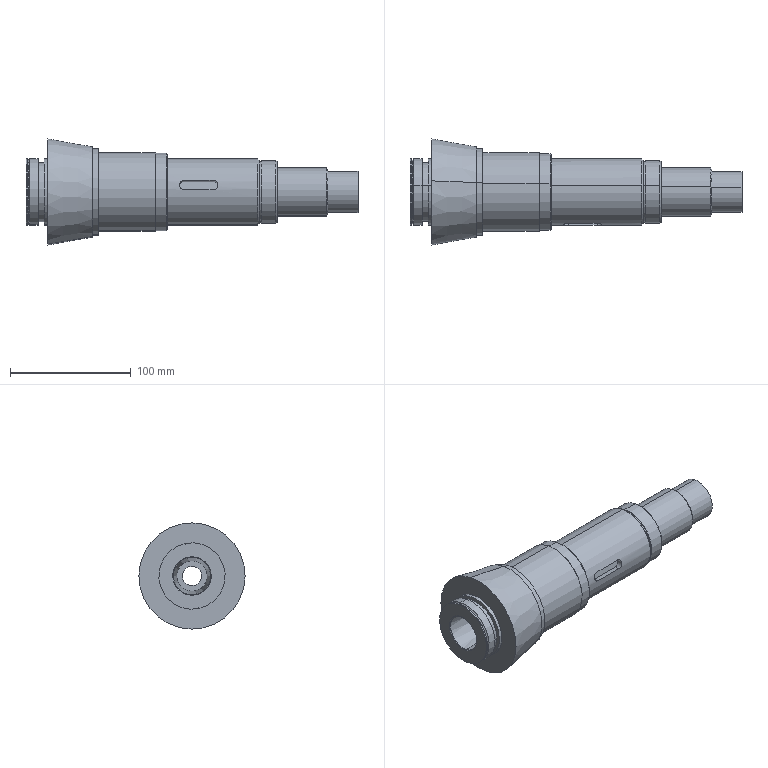Component | SolidWorks | 27Spindle-1 | 1 solid | 75 faces | box 275 x 88 x 88 mm | volume 621740 mm3 | cylinder 33 | plane 21 | cone 17 | torus 4 | commonest cylinder face diameters 55 x8 64 x3 16 x2 28 x2 34 x2 40 x2 52 x2 50 x2
build123d program:
from build123d import *
from OCP.BRepFilletAPI import BRepFilletAPI_MakeChamfer

# Parameters (mm, degrees)
SKETCH27_R           = 27.5
BOSS_EXTRUDE15_DEPTH = 10
SKETCH28_R           = 24.5
BOSS_EXTRUDE16_DEPTH = 5
SKETCH29_R           = 27.5
BOSS_EXTRUDE17_DEPTH = 3
SKETCH30_R           = 44
BOSS_EXTRUDE18_DEPTH = 37
BOSS_EXTRUDE18_TAPER = 10
SKETCH31_R           = 36
BOSS_EXTRUDE19_DEPTH = 5
SKETCH32_R           = 32.5
BOSS_EXTRUDE20_DEPTH = 47
SKETCH33_R           = 32
BOSS_EXTRUDE21_DEPTH = 10
BOSS_EXTRUDE22_START = -57
SKETCH34_R           = 27.5
BOSS_EXTRUDE22_DEPTH = 133
SKETCH35_R           = 25
BOSS_EXTRUDE23_DEPTH = 2
SKETCH36_R           = 26
BOSS_EXTRUDE24_DEPTH = 13
SKETCH37_R           = 20
BOSS_EXTRUDE25_DEPTH = 42
BOSS_EXTRUDE26_START = -250
SKETCH38_R           = 17
BOSS_EXTRUDE26_DEPTH = 275
SKETCH43_R           = 8
CUT_EXTRUDE3_DEPTH   = 180.154
CHAMFER1_SIZE        = 0.5
CHAMFER1_SIZE2       = 0.5164
CHAMFER2_SIZE        = 1
CUT_SWEEP1_PROFILE_R = 1
CUT_EXTRUDE4_DEPTH   = 4
CUT_EXTRUDE5_START   = -27.5
CUT_EXTRUDE5_DEPTH   = 5


with BuildPart() as part:
    # Sketch27 → Boss-Extrude15 (new body)
    with BuildSketch(Plane(origin=(0, 0, 0), x_dir=(0, 0, -1), z_dir=(1, 0, 0))):
        Circle(SKETCH27_R)
    extrude(amount=BOSS_EXTRUDE15_DEPTH)

    # Sketch28 → Boss-Extrude16 (add)
    with BuildSketch(Plane(origin=(10, 0, 0), x_dir=(0, 0, -1), z_dir=(1, 0, 0))):
        Circle(SKETCH28_R)
    extrude(amount=BOSS_EXTRUDE16_DEPTH)

    # Sketch29 → Boss-Extrude17 (add)
    with BuildSketch(Plane(origin=(15, 0, 0), x_dir=(0, 0, -1), z_dir=(1, 0, 0))):
        Circle(SKETCH29_R)
    extrude(amount=BOSS_EXTRUDE17_DEPTH)

    # Sketch30 → Boss-Extrude18 (add)
    with BuildSketch(Plane(origin=(18, 0, 0), x_dir=(0, 0, -1), z_dir=(1, 0, 0))):
        Circle(SKETCH30_R)
    extrude(amount=BOSS_EXTRUDE18_DEPTH, taper=BOSS_EXTRUDE18_TAPER)

    # Sketch31 → Boss-Extrude19 (add)
    with BuildSketch(Plane(origin=(55, 0, 0), x_dir=(0, 0, -1), z_dir=(1, 0, 0))):
        Circle(SKETCH31_R)
    extrude(amount=BOSS_EXTRUDE19_DEPTH)

    # Sketch32 → Boss-Extrude20 (add)
    with BuildSketch(Plane(origin=(60, 0, 0), x_dir=(0, 0, -1), z_dir=(1, 0, 0))):
        Circle(SKETCH32_R)
    extrude(amount=BOSS_EXTRUDE20_DEPTH)

    # Sketch33 → Boss-Extrude21 (add)
    with BuildSketch(Plane(origin=(107, 0, 0), x_dir=(0, 0, -1), z_dir=(1, 0, 0))):
        Circle(SKETCH33_R)
    extrude(amount=BOSS_EXTRUDE21_DEPTH)

    # Sketch34 → Boss-Extrude22 (add)
    with BuildSketch(Plane(origin=(117, 0, 0), x_dir=(0, 0, -1), z_dir=(1, 0, 0)).offset(BOSS_EXTRUDE22_START)):
        Circle(SKETCH34_R)
    extrude(amount=BOSS_EXTRUDE22_DEPTH)

    # Sketch35 → Boss-Extrude23 (add)
    with BuildSketch(Plane(origin=(193, 0, 0), x_dir=(0, 0, -1), z_dir=(1, 0, 0))):
        Circle(SKETCH35_R)
    extrude(amount=BOSS_EXTRUDE23_DEPTH)

    # Sketch36 → Boss-Extrude24 (add)
    with BuildSketch(Plane(origin=(195, 0, 0), x_dir=(0, 0, -1), z_dir=(1, 0, 0))):
        with Locations(Location((0, 0, 0), (0, 0, 180))):
            Circle(SKETCH36_R)
    extrude(amount=BOSS_EXTRUDE24_DEPTH)

    # Sketch37 → Boss-Extrude25 (add)
    with BuildSketch(Plane(origin=(208, 0, 0), x_dir=(0, 0, -1), z_dir=(1, 0, 0))):
        with Locations(Location((0, 0, 0), (0, 0, 180))):
            Circle(SKETCH37_R)
    extrude(amount=BOSS_EXTRUDE25_DEPTH)

    # Sketch38 → Boss-Extrude26 (add)
    with BuildSketch(Plane(origin=(250, 0, 0), x_dir=(0, 0, -1), z_dir=(1, 0, 0)).offset(BOSS_EXTRUDE26_START)):
        Circle(SKETCH38_R)
    extrude(amount=BOSS_EXTRUDE26_DEPTH)

    # Sketch42 → Cut-Revolve1 (revolve, cut)
    with BuildSketch(Plane(origin=(0, 0, 0), x_dir=(1, 0, 0), z_dir=(0, 1, 0)), mode=Mode.PRIVATE) as cut_revolve1_sk:
        Polygon((0, 0), (0, 15.5), (92, 12.625), (92, 14), (107, 14), (107, 0), align=None)
    revolve(cut_revolve1_sk.sketch.rotate(Axis((-73.512, 0, 0), (1, 0, 0)), 180), axis=Axis((-73.512, 0, 0), (1, 0, 0)), mode=Mode.SUBTRACT)

    # Sketch43 → Cut-Extrude3 (cut, through all)
    with BuildSketch(Plane.ZY.offset(-107)):
        Circle(SKETCH43_R)
    extrude(amount=-CUT_EXTRUDE3_DEPTH, mode=Mode.SUBTRACT)

    # Chamfer1: one chamfer whose edges measure the first distance from different faces: ONE call of the kernel's chamfer builder (chamfer() names one face for all edges)
    chamfer1_edges_1 = [part.edges().sort_by_distance(p)[0] for p in [
        (0, 0, -15.5),
    ]]
    chamfer1_side_1 = [part.faces().sort_by_distance(p)[0] for p in [
        (0, 0, 26.722),
    ]]
    chamfer1_edges_2 = [part.edges().sort_by_distance(p)[0] for p in [
        (275, 0, -8),
    ]]
    chamfer1 = BRepFilletAPI_MakeChamfer(part.part.solid().wrapped)
    for e in chamfer1_edges_1:
        chamfer1.Add(CHAMFER1_SIZE, CHAMFER1_SIZE2, e.wrapped, chamfer1_side_1[0].wrapped)  # the first distance lies on this face
    for e in chamfer1_edges_2:
        chamfer1.Add(CHAMFER1_SIZE, e.wrapped)
    add(Compound.cast(chamfer1.Shape()), mode=Mode.REPLACE)

    # Chamfer2
    chamfer2_edges = [part.edges().sort_by_distance(p)[0] for p in [
        (117, 0, 32),
        (193, 0, 27.5),
        (208, 0, -26),
        (250, 0, -20),
    ]]
    chamfer(chamfer2_edges, length=CHAMFER2_SIZE)

    # Cut-Sweep1: sweep along a path in Sketch44
    with BuildLine(Plane.ZY.offset(-2)) as cut_sweep1_path:
        CenterArc((0, 0), 27.5, 0, 360)
    # Cut-Sweep1 profile (on start of the path) → Cut-Sweep1 (sweep, cut)
    with BuildSketch(Plane(origin=(2, 0, 27.5), x_dir=(0, 0, 1), z_dir=(0, 1, 0))):
        Circle(CUT_SWEEP1_PROFILE_R)
    sweep(path=cut_sweep1_path.line, mode=Mode.SUBTRACT)

    # Sketch57 → Cut-Extrude4 (cut, symmetric)
    with BuildSketch(Plane.XY):
        with BuildLine():
            Line((92.495, 22.5), (169.972, 22.5))
            ThreePointArc((169.972, 22.5), (179.326, 23.773), (188, 27.5))
            Line((188, 27.5), (188, 32.5))
            Line((188, 32.5), (68, 32.5))
            ThreePointArc((68, 32.5), (79.266, 25.096), (92.495, 22.5))
        make_face()
    extrude(amount=CUT_EXTRUDE4_DEPTH, both=True, mode=Mode.SUBTRACT)

    # Sketch58 → Cut-Extrude5 (cut)
    with BuildSketch(Plane(origin=(0, 0, 0), x_dir=(1, 0, 0), z_dir=(0, 1, 0)).offset(CUT_EXTRUDE5_START)):
        with BuildLine():
            Line((131, 4), (155, 4))
            ThreePointArc((155, 4), (159, 0), (155, -4))
            Line((155, -4), (131, -4))
            ThreePointArc((131, -4), (127, 0), (131, 4))
        make_face()
    extrude(amount=CUT_EXTRUDE5_DEPTH, mode=Mode.SUBTRACT)


solid = part.part

# Placed as in the assembly
solid = solid.moved(Location((-120.043, 1.776, 250), (-12, 0, 0)))